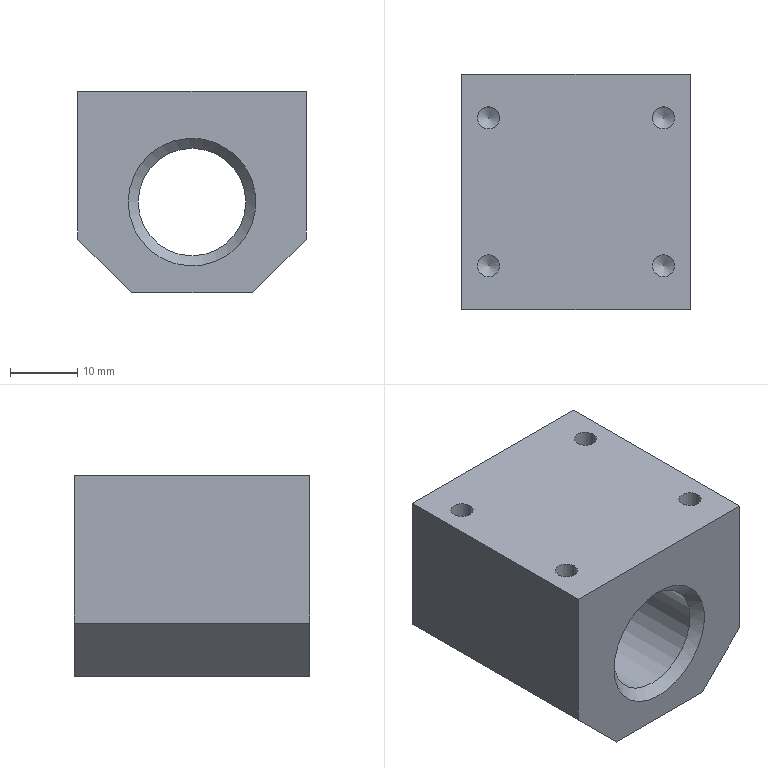Component | NX | SLIDE_NUT | 1 solid | 19 faces | volume 25881 mm3 | plane 8 | cone 6 | cylinder 5 | commonest cylinder face diameters 3.3 x4 16 x1